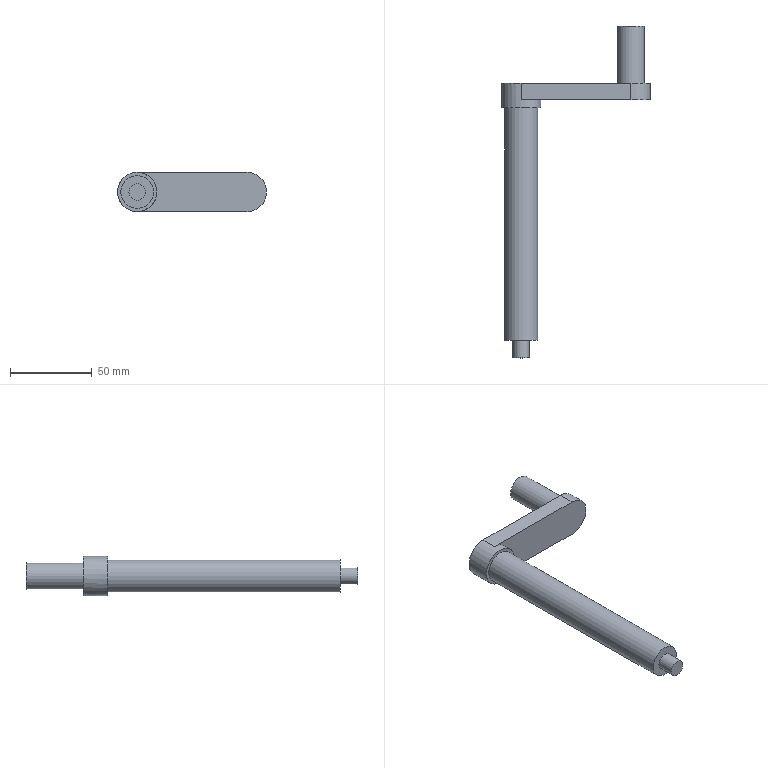Component | NX | ROCKER | 1 solid | 13 faces | box 91 x 202.7 x 24 mm | volume 75353 mm3 | plane 8 | cylinder 5 | commonest cylinder face diameters 24 x2 10 x1 20 x1 16 x1
STEP:
#1=CARTESIAN_POINT('',(0.,0.,0.));
#2=DIRECTION('',(0.,0.,1.));
#3=DIRECTION('',(1.,0.,0.));
#4=AXIS2_PLACEMENT_3D('',#1,#2,#3);
#5=CARTESIAN_POINT('',(-114.826,125.,90.));
#6=VERTEX_POINT('',#5);
#7=CARTESIAN_POINT('',(-126.826,125.,102.));
#8=VERTEX_POINT('',#7);
#9=CARTESIAN_POINT('',(-126.826,125.,90.));
#10=DIRECTION('',(0.,1.,0.));
#11=DIRECTION('',(1.,0.,0.));
#12=AXIS2_PLACEMENT_3D('',#9,#10,#11);
#13=CIRCLE('',#12,12.);
#14=CARTESIAN_POINT('',(-126.826,139.995,90.));
#15=DIRECTION('',(0.,-1.,0.));
#16=DIRECTION('',(-1.,0.,0.));
#17=AXIS2_PLACEMENT_3D('',#14,#15,#16);
#18=CYLINDRICAL_SURFACE('',#17,12.);
#19=CARTESIAN_POINT('',(9.425,14.995));
#20=DIRECTION('',(-1.,0.));
#21=VECTOR('',#20,1.);
#22=LINE('',#19,#21);
#23=(GEOMETRIC_REPRESENTATION_CONTEXT(2)PARAMETRIC_REPRESENTATION_CONTEXT()REPRESENTATION_CONTEXT('',''));
#24=DEFINITIONAL_REPRESENTATION('',(#22),#23);
#25=PCURVE('',#18,#24);
#26=CARTESIAN_POINT('',(-126.826,125.,90.));
#27=DIRECTION('',(0.,1.,0.));
#28=DIRECTION('',(1.,0.,0.));
#29=AXIS2_PLACEMENT_3D('',#26,#27,#28);
#30=PLANE('',#29);
#31=CARTESIAN_POINT('',(0.,0.));
#32=DIRECTION('',(1.,0.));
#33=AXIS2_PLACEMENT_2D('',#31,#32);
#34=CIRCLE('',#33,12.);
#35=(GEOMETRIC_REPRESENTATION_CONTEXT(2)PARAMETRIC_REPRESENTATION_CONTEXT()REPRESENTATION_CONTEXT('',''));
#36=DEFINITIONAL_REPRESENTATION('',(#34),#35);
#37=PCURVE('',#30,#36);
#38=SURFACE_CURVE('',#13,(#25,#37),.PCURVE_S1.);
#39=EDGE_CURVE('',#6,#8,#38,.T.);
#40=ORIENTED_EDGE('',*,*,#39,.T.);
#41=CARTESIAN_POINT('',(-126.826,129.995,102.));
#42=VERTEX_POINT('',#41);
#43=CARTESIAN_POINT('',(-126.826,129.995,102.));
#44=CARTESIAN_POINT('',(-126.826,125.,102.));
#45=B_SPLINE_CURVE_WITH_KNOTS('',1,(#43,#44),.UNSPECIFIED.,.F.,.F.,(2,2),(10.,14.995),.PIECEWISE_BEZIER_KNOTS.);
#46=CARTESIAN_POINT('',(4.712,0.));
#47=DIRECTION('',(0.,1.));
#48=VECTOR('',#47,1.);
#49=LINE('',#46,#48);
#50=(GEOMETRIC_REPRESENTATION_CONTEXT(2)PARAMETRIC_REPRESENTATION_CONTEXT()REPRESENTATION_CONTEXT('',''));
#51=DEFINITIONAL_REPRESENTATION('',(#49),#50);
#52=PCURVE('',#18,#51);
#53=CARTESIAN_POINT('',(10.996,0.));
#54=DIRECTION('',(0.,1.));
#55=VECTOR('',#54,1.);
#56=LINE('',#53,#55);
#57=(GEOMETRIC_REPRESENTATION_CONTEXT(2)PARAMETRIC_REPRESENTATION_CONTEXT()REPRESENTATION_CONTEXT('',''));
#58=DEFINITIONAL_REPRESENTATION('',(#56),#57);
#59=PCURVE('',#18,#58);
#60=SEAM_CURVE('',#45,(#52,#59),.PCURVE_S1.);
#61=EDGE_CURVE('',#42,#8,#60,.T.);
#62=ORIENTED_EDGE('',*,*,#61,.F.);
#63=CARTESIAN_POINT('',(-126.826,139.995,102.));
#64=VERTEX_POINT('',#63);
#65=CARTESIAN_POINT('',(-126.826,139.995,102.));
#66=DIRECTION('',(0.,-1.,0.));
#67=VECTOR('',#66,1.);
#68=LINE('',#65,#67);
#69=CARTESIAN_POINT('',(4.712,0.));
#70=DIRECTION('',(0.,1.));
#71=VECTOR('',#70,1.);
#72=LINE('',#69,#71);
#73=(GEOMETRIC_REPRESENTATION_CONTEXT(2)PARAMETRIC_REPRESENTATION_CONTEXT()REPRESENTATION_CONTEXT('',''));
#74=DEFINITIONAL_REPRESENTATION('',(#72),#73);
#75=PCURVE('',#18,#74);
#76=CARTESIAN_POINT('',(-126.826,139.995,102.));
#77=DIRECTION('',(0.,0.,-1.));
#78=DIRECTION('',(0.,1.,0.));
#79=AXIS2_PLACEMENT_3D('',#76,#77,#78);
#80=PLANE('',#79);
#81=CARTESIAN_POINT('',(0.,0.));
#82=DIRECTION('',(-1.,0.));
#83=VECTOR('',#82,1.);
#84=LINE('',#81,#83);
#85=(GEOMETRIC_REPRESENTATION_CONTEXT(2)PARAMETRIC_REPRESENTATION_CONTEXT()REPRESENTATION_CONTEXT('',''));
#86=DEFINITIONAL_REPRESENTATION('',(#84),#85);
#87=PCURVE('',#80,#86);
#88=SURFACE_CURVE('',#68,(#75,#87),.PCURVE_S1.);
#89=EDGE_CURVE('',#64,#42,#88,.T.);
#90=ORIENTED_EDGE('',*,*,#89,.F.);
#91=CARTESIAN_POINT('',(-126.826,139.995,78.));
#92=VERTEX_POINT('',#91);
#93=CARTESIAN_POINT('',(-126.826,139.995,90.));
#94=DIRECTION('',(0.,1.,0.));
#95=DIRECTION('',(1.,0.,0.));
#96=AXIS2_PLACEMENT_3D('',#93,#94,#95);
#97=CIRCLE('',#96,12.);
#98=CARTESIAN_POINT('',(9.425,0.));
#99=DIRECTION('',(-1.,0.));
#100=VECTOR('',#99,1.);
#101=LINE('',#98,#100);
#102=(GEOMETRIC_REPRESENTATION_CONTEXT(2)PARAMETRIC_REPRESENTATION_CONTEXT()REPRESENTATION_CONTEXT('',''));
#103=DEFINITIONAL_REPRESENTATION('',(#101),#102);
#104=PCURVE('',#18,#103);
#105=CARTESIAN_POINT('',(-126.826,139.995,90.));
#106=DIRECTION('',(0.,1.,0.));
#107=DIRECTION('',(1.,0.,0.));
#108=AXIS2_PLACEMENT_3D('',#105,#106,#107);
#109=PLANE('',#108);
#110=CARTESIAN_POINT('',(0.,0.));
#111=DIRECTION('',(1.,0.));
#112=AXIS2_PLACEMENT_2D('',#110,#111);
#113=CIRCLE('',#112,12.);
#114=(GEOMETRIC_REPRESENTATION_CONTEXT(2)PARAMETRIC_REPRESENTATION_CONTEXT()REPRESENTATION_CONTEXT('',''));
#115=DEFINITIONAL_REPRESENTATION('',(#113),#114);
#116=PCURVE('',#109,#115);
#117=SURFACE_CURVE('',#97,(#104,#116),.PCURVE_S1.);
#118=EDGE_CURVE('',#92,#64,#117,.T.);
#119=ORIENTED_EDGE('',*,*,#118,.F.);
#120=CARTESIAN_POINT('',(-126.826,129.995,78.));
#121=VERTEX_POINT('',#120);
#122=CARTESIAN_POINT('',(-126.826,139.995,78.));
#123=DIRECTION('',(0.,-1.,0.));
#124=VECTOR('',#123,1.);
#125=LINE('',#122,#124);
#126=CARTESIAN_POINT('',(7.854,0.));
#127=DIRECTION('',(0.,1.));
#128=VECTOR('',#127,1.);
#129=LINE('',#126,#128);
#130=(GEOMETRIC_REPRESENTATION_CONTEXT(2)PARAMETRIC_REPRESENTATION_CONTEXT()REPRESENTATION_CONTEXT('',''));
#131=DEFINITIONAL_REPRESENTATION('',(#129),#130);
#132=PCURVE('',#18,#131);
#133=CARTESIAN_POINT('',(-59.827,139.995,78.));
#134=DIRECTION('',(0.,0.,1.));
#135=DIRECTION('',(0.,-1.,0.));
#136=AXIS2_PLACEMENT_3D('',#133,#134,#135);
#137=PLANE('',#136);
#138=CARTESIAN_POINT('',(0.,-67.));
#139=DIRECTION('',(1.,0.));
#140=VECTOR('',#139,1.);
#141=LINE('',#138,#140);
#142=(GEOMETRIC_REPRESENTATION_CONTEXT(2)PARAMETRIC_REPRESENTATION_CONTEXT()REPRESENTATION_CONTEXT('',''));
#143=DEFINITIONAL_REPRESENTATION('',(#141),#142);
#144=PCURVE('',#137,#143);
#145=SURFACE_CURVE('',#125,(#132,#144),.PCURVE_S1.);
#146=EDGE_CURVE('',#92,#121,#145,.T.);
#147=ORIENTED_EDGE('',*,*,#146,.T.);
#148=CARTESIAN_POINT('',(-126.826,129.995,90.));
#149=DIRECTION('',(0.,-1.,0.));
#150=DIRECTION('',(1.,0.,0.));
#151=AXIS2_PLACEMENT_3D('',#148,#149,#150);
#152=CIRCLE('',#151,12.);
#153=CARTESIAN_POINT('',(3.142,10.));
#154=DIRECTION('',(1.,0.));
#155=VECTOR('',#154,1.);
#156=LINE('',#153,#155);
#157=(GEOMETRIC_REPRESENTATION_CONTEXT(2)PARAMETRIC_REPRESENTATION_CONTEXT()REPRESENTATION_CONTEXT('',''));
#158=DEFINITIONAL_REPRESENTATION('',(#156),#157);
#159=PCURVE('',#18,#158);
#160=CARTESIAN_POINT('',(-126.826,129.995,90.));
#161=DIRECTION('',(0.,-1.,0.));
#162=DIRECTION('',(-1.,0.,0.));
#163=AXIS2_PLACEMENT_3D('',#160,#161,#162);
#164=PLANE('',#163);
#165=CARTESIAN_POINT('',(0.,0.));
#166=DIRECTION('',(-1.,0.));
#167=AXIS2_PLACEMENT_2D('',#165,#166);
#168=CIRCLE('',#167,12.);
#169=(GEOMETRIC_REPRESENTATION_CONTEXT(2)PARAMETRIC_REPRESENTATION_CONTEXT()REPRESENTATION_CONTEXT('',''));
#170=DEFINITIONAL_REPRESENTATION('',(#168),#169);
#171=PCURVE('',#164,#170);
#172=SURFACE_CURVE('',#152,(#159,#171),.PCURVE_S1.);
#173=EDGE_CURVE('',#121,#42,#172,.T.);
#174=ORIENTED_EDGE('',*,*,#173,.T.);
#175=ORIENTED_EDGE('',*,*,#61,.T.);
#176=CARTESIAN_POINT('',(-126.826,125.,90.));
#177=DIRECTION('',(0.,1.,0.));
#178=DIRECTION('',(1.,0.,0.));
#179=AXIS2_PLACEMENT_3D('',#176,#177,#178);
#180=CIRCLE('',#179,12.);
#181=CARTESIAN_POINT('',(15.708,14.995));
#182=DIRECTION('',(-1.,0.));
#183=VECTOR('',#182,1.);
#184=LINE('',#181,#183);
#185=(GEOMETRIC_REPRESENTATION_CONTEXT(2)PARAMETRIC_REPRESENTATION_CONTEXT()REPRESENTATION_CONTEXT('',''));
#186=DEFINITIONAL_REPRESENTATION('',(#184),#185);
#187=PCURVE('',#18,#186);
#188=CARTESIAN_POINT('',(0.,0.));
#189=DIRECTION('',(1.,0.));
#190=AXIS2_PLACEMENT_2D('',#188,#189);
#191=CIRCLE('',#190,12.);
#192=(GEOMETRIC_REPRESENTATION_CONTEXT(2)PARAMETRIC_REPRESENTATION_CONTEXT()REPRESENTATION_CONTEXT('',''));
#193=DEFINITIONAL_REPRESENTATION('',(#191),#192);
#194=PCURVE('',#30,#193);
#195=SURFACE_CURVE('',#180,(#187,#194),.PCURVE_S1.);
#196=EDGE_CURVE('',#8,#6,#195,.T.);
#197=ORIENTED_EDGE('',*,*,#196,.T.);
#198=EDGE_LOOP('',(#40,#62,#90,#119,#147,#174,#175,#197));
#199=FACE_BOUND('',#198,.T.);
#200=ADVANCED_FACE('',(#199),#18,.T.);
#201=CARTESIAN_POINT('',(-121.826,-27.705,90.));
#202=VERTEX_POINT('',#201);
#203=CARTESIAN_POINT('',(-126.826,-27.705,90.));
#204=DIRECTION('',(0.,1.,0.));
#205=DIRECTION('',(1.,0.,0.));
#206=AXIS2_PLACEMENT_3D('',#203,#204,#205);
#207=CIRCLE('',#206,5.);
#208=CARTESIAN_POINT('',(-126.826,-27.705,90.));
#209=DIRECTION('',(0.,-1.,0.));
#210=DIRECTION('',(-1.,0.,0.));
#211=AXIS2_PLACEMENT_3D('',#208,#209,#210);
#212=PLANE('',#211);
#213=CARTESIAN_POINT('',(-5.,0.));
#214=CARTESIAN_POINT('',(-5.,8.66));
#215=CARTESIAN_POINT('',(2.5,4.33));
#216=CARTESIAN_POINT('',(10.,0.));
#217=CARTESIAN_POINT('',(2.5,-4.33));
#218=CARTESIAN_POINT('',(-5.,-8.66));
#219=CARTESIAN_POINT('',(-5.,0.));
#220=(BOUNDED_CURVE()B_SPLINE_CURVE(2,(#213,#214,#215,#216,#217,#218,#219),.UNSPECIFIED.,.T.,.F.)B_SPLINE_CURVE_WITH_KNOTS((1,2,2,2,2,1),(-2.094,0.,2.094,4.189,6.283,8.378),.UNSPECIFIED.)CURVE()GEOMETRIC_REPRESENTATION_ITEM()RATIONAL_B_SPLINE_CURVE((1.,0.5,1.,0.5,1.,0.5,1.))REPRESENTATION_ITEM(''));
#221=(GEOMETRIC_REPRESENTATION_CONTEXT(2)PARAMETRIC_REPRESENTATION_CONTEXT()REPRESENTATION_CONTEXT('',''));
#222=DEFINITIONAL_REPRESENTATION('',(#220),#221);
#223=PCURVE('',#212,#222);
#224=CARTESIAN_POINT('',(-126.826,-27.705,90.));
#225=DIRECTION('',(0.,1.,0.));
#226=DIRECTION('',(1.,0.,0.));
#227=AXIS2_PLACEMENT_3D('',#224,#225,#226);
#228=CYLINDRICAL_SURFACE('',#227,5.);
#229=CARTESIAN_POINT('',(0.,0.));
#230=DIRECTION('',(1.,0.));
#231=VECTOR('',#230,1.);
#232=LINE('',#229,#231);
#233=(GEOMETRIC_REPRESENTATION_CONTEXT(2)PARAMETRIC_REPRESENTATION_CONTEXT()REPRESENTATION_CONTEXT('',''));
#234=DEFINITIONAL_REPRESENTATION('',(#232),#233);
#235=PCURVE('',#228,#234);
#236=SURFACE_CURVE('',#207,(#223,#235),.PCURVE_S1.);
#237=EDGE_CURVE('',#202,#202,#236,.T.);
#238=ORIENTED_EDGE('',*,*,#237,.F.);
#239=EDGE_LOOP('',(#238));
#240=FACE_BOUND('',#239,.T.);
#241=ADVANCED_FACE('',(#240),#212,.T.);
#242=CARTESIAN_POINT('',(-121.826,-17.005,90.));
#243=VERTEX_POINT('',#242);
#244=CARTESIAN_POINT('',(-126.826,-17.005,90.));
#245=DIRECTION('',(0.,-1.,0.));
#246=DIRECTION('',(1.,0.,0.));
#247=AXIS2_PLACEMENT_3D('',#244,#245,#246);
#248=CIRCLE('',#247,5.);
#249=CARTESIAN_POINT('',(6.283,10.7));
#250=DIRECTION('',(-1.,0.));
#251=VECTOR('',#250,1.);
#252=LINE('',#249,#251);
#253=(GEOMETRIC_REPRESENTATION_CONTEXT(2)PARAMETRIC_REPRESENTATION_CONTEXT()REPRESENTATION_CONTEXT('',''));
#254=DEFINITIONAL_REPRESENTATION('',(#252),#253);
#255=PCURVE('',#228,#254);
#256=CARTESIAN_POINT('',(-126.826,-17.005,90.));
#257=DIRECTION('',(0.,-1.,0.));
#258=DIRECTION('',(-1.,0.,0.));
#259=AXIS2_PLACEMENT_3D('',#256,#257,#258);
#260=PLANE('',#259);
#261=CARTESIAN_POINT('',(0.,0.));
#262=DIRECTION('',(-1.,0.));
#263=AXIS2_PLACEMENT_2D('',#261,#262);
#264=CIRCLE('',#263,5.);
#265=(GEOMETRIC_REPRESENTATION_CONTEXT(2)PARAMETRIC_REPRESENTATION_CONTEXT()REPRESENTATION_CONTEXT('',''));
#266=DEFINITIONAL_REPRESENTATION('',(#264),#265);
#267=PCURVE('',#260,#266);
#268=SURFACE_CURVE('',#248,(#255,#267),.PCURVE_S1.);
#269=EDGE_CURVE('',#243,#243,#268,.T.);
#270=ORIENTED_EDGE('',*,*,#269,.T.);
#271=CARTESIAN_POINT('',(-121.826,-27.705,90.));
#272=CARTESIAN_POINT('',(-121.826,-17.005,90.));
#273=B_SPLINE_CURVE_WITH_KNOTS('',1,(#271,#272),.UNSPECIFIED.,.F.,.F.,(2,2),(0.,10.7),.PIECEWISE_BEZIER_KNOTS.);
#274=CARTESIAN_POINT('',(0.,0.));
#275=DIRECTION('',(0.,1.));
#276=VECTOR('',#275,1.);
#277=LINE('',#274,#276);
#278=(GEOMETRIC_REPRESENTATION_CONTEXT(2)PARAMETRIC_REPRESENTATION_CONTEXT()REPRESENTATION_CONTEXT('',''));
#279=DEFINITIONAL_REPRESENTATION('',(#277),#278);
#280=PCURVE('',#228,#279);
#281=CARTESIAN_POINT('',(6.283,0.));
#282=DIRECTION('',(0.,1.));
#283=VECTOR('',#282,1.);
#284=LINE('',#281,#283);
#285=(GEOMETRIC_REPRESENTATION_CONTEXT(2)PARAMETRIC_REPRESENTATION_CONTEXT()REPRESENTATION_CONTEXT('',''));
#286=DEFINITIONAL_REPRESENTATION('',(#284),#285);
#287=PCURVE('',#228,#286);
#288=SEAM_CURVE('',#273,(#280,#287),.PCURVE_S1.);
#289=EDGE_CURVE('',#202,#243,#288,.T.);
#290=ORIENTED_EDGE('',*,*,#289,.F.);
#291=ORIENTED_EDGE('',*,*,#237,.T.);
#292=ORIENTED_EDGE('',*,*,#289,.T.);
#293=EDGE_LOOP('',(#270,#290,#291,#292));
#294=FACE_BOUND('',#293,.T.);
#295=ADVANCED_FACE('',(#294),#228,.T.);
#296=ORIENTED_EDGE('',*,*,#269,.F.);
#297=EDGE_LOOP('',(#296));
#298=FACE_BOUND('',#297,.T.);
#299=CARTESIAN_POINT('',(-116.826,-17.005,90.));
#300=VERTEX_POINT('',#299);
#301=CARTESIAN_POINT('',(-126.826,-17.005,90.));
#302=DIRECTION('',(0.,1.,0.));
#303=DIRECTION('',(1.,0.,0.));
#304=AXIS2_PLACEMENT_3D('',#301,#302,#303);
#305=CIRCLE('',#304,10.);
#306=CARTESIAN_POINT('',(-10.,0.));
#307=CARTESIAN_POINT('',(-10.,17.321));
#308=CARTESIAN_POINT('',(5.,8.66));
#309=CARTESIAN_POINT('',(20.,0.));
#310=CARTESIAN_POINT('',(5.,-8.66));
#311=CARTESIAN_POINT('',(-10.,-17.321));
#312=CARTESIAN_POINT('',(-10.,0.));
#313=(BOUNDED_CURVE()B_SPLINE_CURVE(2,(#306,#307,#308,#309,#310,#311,#312),.UNSPECIFIED.,.T.,.F.)B_SPLINE_CURVE_WITH_KNOTS((1,2,2,2,2,1),(-2.094,0.,2.094,4.189,6.283,8.378),.UNSPECIFIED.)CURVE()GEOMETRIC_REPRESENTATION_ITEM()RATIONAL_B_SPLINE_CURVE((1.,0.5,1.,0.5,1.,0.5,1.))REPRESENTATION_ITEM(''));
#314=(GEOMETRIC_REPRESENTATION_CONTEXT(2)PARAMETRIC_REPRESENTATION_CONTEXT()REPRESENTATION_CONTEXT('',''));
#315=DEFINITIONAL_REPRESENTATION('',(#313),#314);
#316=PCURVE('',#260,#315);
#317=CARTESIAN_POINT('',(-126.826,-17.005,90.));
#318=DIRECTION('',(0.,1.,0.));
#319=DIRECTION('',(1.,0.,0.));
#320=AXIS2_PLACEMENT_3D('',#317,#318,#319);
#321=CYLINDRICAL_SURFACE('',#320,10.);
#322=CARTESIAN_POINT('',(0.,0.));
#323=DIRECTION('',(1.,0.));
#324=VECTOR('',#323,1.);
#325=LINE('',#322,#324);
#326=(GEOMETRIC_REPRESENTATION_CONTEXT(2)PARAMETRIC_REPRESENTATION_CONTEXT()REPRESENTATION_CONTEXT('',''));
#327=DEFINITIONAL_REPRESENTATION('',(#325),#326);
#328=PCURVE('',#321,#327);
#329=SURFACE_CURVE('',#305,(#316,#328),.PCURVE_S1.);
#330=EDGE_CURVE('',#300,#300,#329,.T.);
#331=ORIENTED_EDGE('',*,*,#330,.F.);
#332=EDGE_LOOP('',(#331));
#333=FACE_BOUND('',#332,.T.);
#334=ADVANCED_FACE('',(#298,#333),#260,.T.);
#335=CARTESIAN_POINT('',(-116.826,125.,90.));
#336=VERTEX_POINT('',#335);
#337=CARTESIAN_POINT('',(-126.826,125.,90.));
#338=DIRECTION('',(0.,-1.,0.));
#339=DIRECTION('',(1.,0.,0.));
#340=AXIS2_PLACEMENT_3D('',#337,#338,#339);
#341=CIRCLE('',#340,10.);
#342=CARTESIAN_POINT('',(6.283,142.005));
#343=DIRECTION('',(-1.,0.));
#344=VECTOR('',#343,1.);
#345=LINE('',#342,#344);
#346=(GEOMETRIC_REPRESENTATION_CONTEXT(2)PARAMETRIC_REPRESENTATION_CONTEXT()REPRESENTATION_CONTEXT('',''));
#347=DEFINITIONAL_REPRESENTATION('',(#345),#346);
#348=PCURVE('',#321,#347);
#349=CARTESIAN_POINT('',(10.,0.));
#350=CARTESIAN_POINT('',(10.,-17.321));
#351=CARTESIAN_POINT('',(-5.,-8.66));
#352=CARTESIAN_POINT('',(-20.,-0.));
#353=CARTESIAN_POINT('',(-5.,8.66));
#354=CARTESIAN_POINT('',(10.,17.321));
#355=CARTESIAN_POINT('',(10.,0.));
#356=(BOUNDED_CURVE()B_SPLINE_CURVE(2,(#349,#350,#351,#352,#353,#354,#355),.UNSPECIFIED.,.T.,.F.)B_SPLINE_CURVE_WITH_KNOTS((1,2,2,2,2,1),(-2.094,0.,2.094,4.189,6.283,8.378),.UNSPECIFIED.)CURVE()GEOMETRIC_REPRESENTATION_ITEM()RATIONAL_B_SPLINE_CURVE((1.,0.5,1.,0.5,1.,0.5,1.))REPRESENTATION_ITEM(''));
#357=(GEOMETRIC_REPRESENTATION_CONTEXT(2)PARAMETRIC_REPRESENTATION_CONTEXT()REPRESENTATION_CONTEXT('',''));
#358=DEFINITIONAL_REPRESENTATION('',(#356),#357);
#359=PCURVE('',#30,#358);
#360=SURFACE_CURVE('',#341,(#348,#359),.PCURVE_S1.);
#361=EDGE_CURVE('',#336,#336,#360,.T.);
#362=ORIENTED_EDGE('',*,*,#361,.T.);
#363=CARTESIAN_POINT('',(-116.826,-17.005,90.));
#364=CARTESIAN_POINT('',(-116.826,125.,90.));
#365=B_SPLINE_CURVE_WITH_KNOTS('',1,(#363,#364),.UNSPECIFIED.,.F.,.F.,(2,2),(0.,142.005),.PIECEWISE_BEZIER_KNOTS.);
#366=CARTESIAN_POINT('',(0.,0.));
#367=DIRECTION('',(0.,1.));
#368=VECTOR('',#367,1.);
#369=LINE('',#366,#368);
#370=(GEOMETRIC_REPRESENTATION_CONTEXT(2)PARAMETRIC_REPRESENTATION_CONTEXT()REPRESENTATION_CONTEXT('',''));
#371=DEFINITIONAL_REPRESENTATION('',(#369),#370);
#372=PCURVE('',#321,#371);
#373=CARTESIAN_POINT('',(6.283,0.));
#374=DIRECTION('',(0.,1.));
#375=VECTOR('',#374,1.);
#376=LINE('',#373,#375);
#377=(GEOMETRIC_REPRESENTATION_CONTEXT(2)PARAMETRIC_REPRESENTATION_CONTEXT()REPRESENTATION_CONTEXT('',''));
#378=DEFINITIONAL_REPRESENTATION('',(#376),#377);
#379=PCURVE('',#321,#378);
#380=SEAM_CURVE('',#365,(#372,#379),.PCURVE_S1.);
#381=EDGE_CURVE('',#300,#336,#380,.T.);
#382=ORIENTED_EDGE('',*,*,#381,.F.);
#383=ORIENTED_EDGE('',*,*,#330,.T.);
#384=ORIENTED_EDGE('',*,*,#381,.T.);
#385=EDGE_LOOP('',(#362,#382,#383,#384));
#386=FACE_BOUND('',#385,.T.);
#387=ADVANCED_FACE('',(#386),#321,.T.);
#388=CARTESIAN_POINT('',(-51.827,139.995,90.));
#389=VERTEX_POINT('',#388);
#390=CARTESIAN_POINT('',(-59.827,139.995,90.));
#391=DIRECTION('',(0.,1.,0.));
#392=DIRECTION('',(1.,0.,0.));
#393=AXIS2_PLACEMENT_3D('',#390,#391,#392);
#394=CIRCLE('',#393,8.);
#395=CARTESIAN_POINT('',(67.,0.));
#396=DIRECTION('',(1.,0.));
#397=AXIS2_PLACEMENT_2D('',#395,#396);
#398=CIRCLE('',#397,8.);
#399=(GEOMETRIC_REPRESENTATION_CONTEXT(2)PARAMETRIC_REPRESENTATION_CONTEXT()REPRESENTATION_CONTEXT('',''));
#400=DEFINITIONAL_REPRESENTATION('',(#398),#399);
#401=PCURVE('',#109,#400);
#402=CARTESIAN_POINT('',(-59.827,139.995,90.));
#403=DIRECTION('',(0.,1.,0.));
#404=DIRECTION('',(1.,0.,0.));
#405=AXIS2_PLACEMENT_3D('',#402,#403,#404);
#406=CYLINDRICAL_SURFACE('',#405,8.);
#407=CARTESIAN_POINT('',(0.,0.));
#408=DIRECTION('',(1.,0.));
#409=VECTOR('',#408,1.);
#410=LINE('',#407,#409);
#411=(GEOMETRIC_REPRESENTATION_CONTEXT(2)PARAMETRIC_REPRESENTATION_CONTEXT()REPRESENTATION_CONTEXT('',''));
#412=DEFINITIONAL_REPRESENTATION('',(#410),#411);
#413=PCURVE('',#406,#412);
#414=SURFACE_CURVE('',#394,(#401,#413),.PCURVE_S1.);
#415=EDGE_CURVE('',#389,#389,#414,.T.);
#416=ORIENTED_EDGE('',*,*,#415,.F.);
#417=EDGE_LOOP('',(#416));
#418=FACE_BOUND('',#417,.T.);
#419=ORIENTED_EDGE('',*,*,#118,.T.);
#420=CARTESIAN_POINT('',(-59.827,139.995,102.));
#421=VERTEX_POINT('',#420);
#422=CARTESIAN_POINT('',(-126.826,139.995,102.));
#423=DIRECTION('',(1.,0.,0.));
#424=VECTOR('',#423,1.);
#425=LINE('',#422,#424);
#426=CARTESIAN_POINT('',(0.,-12.));
#427=DIRECTION('',(1.,0.));
#428=VECTOR('',#427,1.);
#429=LINE('',#426,#428);
#430=(GEOMETRIC_REPRESENTATION_CONTEXT(2)PARAMETRIC_REPRESENTATION_CONTEXT()REPRESENTATION_CONTEXT('',''));
#431=DEFINITIONAL_REPRESENTATION('',(#429),#430);
#432=PCURVE('',#109,#431);
#433=CARTESIAN_POINT('',(0.,0.));
#434=DIRECTION('',(0.,1.));
#435=VECTOR('',#434,1.);
#436=LINE('',#433,#435);
#437=(GEOMETRIC_REPRESENTATION_CONTEXT(2)PARAMETRIC_REPRESENTATION_CONTEXT()REPRESENTATION_CONTEXT('',''));
#438=DEFINITIONAL_REPRESENTATION('',(#436),#437);
#439=PCURVE('',#80,#438);
#440=SURFACE_CURVE('',#425,(#432,#439),.PCURVE_S1.);
#441=EDGE_CURVE('',#64,#421,#440,.T.);
#442=ORIENTED_EDGE('',*,*,#441,.T.);
#443=CARTESIAN_POINT('',(-59.826,139.995,78.));
#444=VERTEX_POINT('',#443);
#445=CARTESIAN_POINT('',(-59.827,139.995,90.));
#446=DIRECTION('',(0.,1.,0.));
#447=DIRECTION('',(1.,0.,0.));
#448=AXIS2_PLACEMENT_3D('',#445,#446,#447);
#449=CIRCLE('',#448,12.);
#450=CARTESIAN_POINT('',(67.,0.));
#451=DIRECTION('',(1.,0.));
#452=AXIS2_PLACEMENT_2D('',#450,#451);
#453=CIRCLE('',#452,12.);
#454=(GEOMETRIC_REPRESENTATION_CONTEXT(2)PARAMETRIC_REPRESENTATION_CONTEXT()REPRESENTATION_CONTEXT('',''));
#455=DEFINITIONAL_REPRESENTATION('',(#453),#454);
#456=PCURVE('',#109,#455);
#457=CARTESIAN_POINT('',(-59.827,139.995,90.));
#458=DIRECTION('',(0.,-1.,0.));
#459=DIRECTION('',(-1.,0.,0.));
#460=AXIS2_PLACEMENT_3D('',#457,#458,#459);
#461=CYLINDRICAL_SURFACE('',#460,12.);
#462=CARTESIAN_POINT('',(9.425,0.));
#463=DIRECTION('',(-1.,0.));
#464=VECTOR('',#463,1.);
#465=LINE('',#462,#464);
#466=(GEOMETRIC_REPRESENTATION_CONTEXT(2)PARAMETRIC_REPRESENTATION_CONTEXT()REPRESENTATION_CONTEXT('',''));
#467=DEFINITIONAL_REPRESENTATION('',(#465),#466);
#468=PCURVE('',#461,#467);
#469=SURFACE_CURVE('',#449,(#456,#468),.PCURVE_S1.);
#470=EDGE_CURVE('',#421,#444,#469,.T.);
#471=ORIENTED_EDGE('',*,*,#470,.T.);
#472=CARTESIAN_POINT('',(-59.827,139.995,78.));
#473=DIRECTION('',(-1.,0.,0.));
#474=VECTOR('',#473,1.);
#475=LINE('',#472,#474);
#476=CARTESIAN_POINT('',(67.,12.));
#477=DIRECTION('',(-1.,0.));
#478=VECTOR('',#477,1.);
#479=LINE('',#476,#478);
#480=(GEOMETRIC_REPRESENTATION_CONTEXT(2)PARAMETRIC_REPRESENTATION_CONTEXT()REPRESENTATION_CONTEXT('',''));
#481=DEFINITIONAL_REPRESENTATION('',(#479),#480);
#482=PCURVE('',#109,#481);
#483=CARTESIAN_POINT('',(0.,0.));
#484=DIRECTION('',(0.,-1.));
#485=VECTOR('',#484,1.);
#486=LINE('',#483,#485);
#487=(GEOMETRIC_REPRESENTATION_CONTEXT(2)PARAMETRIC_REPRESENTATION_CONTEXT()REPRESENTATION_CONTEXT('',''));
#488=DEFINITIONAL_REPRESENTATION('',(#486),#487);
#489=PCURVE('',#137,#488);
#490=SURFACE_CURVE('',#475,(#482,#489),.PCURVE_S1.);
#491=EDGE_CURVE('',#444,#92,#490,.T.);
#492=ORIENTED_EDGE('',*,*,#491,.T.);
#493=EDGE_LOOP('',(#419,#442,#471,#492));
#494=FACE_BOUND('',#493,.T.);
#495=ADVANCED_FACE('',(#418,#494),#109,.T.);
#496=ORIENTED_EDGE('',*,*,#361,.F.);
#497=EDGE_LOOP('',(#496));
#498=FACE_BOUND('',#497,.T.);
#499=ORIENTED_EDGE('',*,*,#39,.F.);
#500=ORIENTED_EDGE('',*,*,#196,.F.);
#501=EDGE_LOOP('',(#499,#500));
#502=FACE_BOUND('',#501,.T.);
#503=ADVANCED_FACE('',(#498,#502),#30,.F.);
#504=CARTESIAN_POINT('',(-59.827,129.995,102.));
#505=VERTEX_POINT('',#504);
#506=CARTESIAN_POINT('',(-126.826,129.995,102.));
#507=DIRECTION('',(1.,0.,0.));
#508=VECTOR('',#507,1.);
#509=LINE('',#506,#508);
#510=CARTESIAN_POINT('',(-10.,0.));
#511=DIRECTION('',(0.,1.));
#512=VECTOR('',#511,1.);
#513=LINE('',#510,#512);
#514=(GEOMETRIC_REPRESENTATION_CONTEXT(2)PARAMETRIC_REPRESENTATION_CONTEXT()REPRESENTATION_CONTEXT('',''));
#515=DEFINITIONAL_REPRESENTATION('',(#513),#514);
#516=PCURVE('',#80,#515);
#517=CARTESIAN_POINT('',(0.,-12.));
#518=DIRECTION('',(-1.,0.));
#519=VECTOR('',#518,1.);
#520=LINE('',#517,#519);
#521=(GEOMETRIC_REPRESENTATION_CONTEXT(2)PARAMETRIC_REPRESENTATION_CONTEXT()REPRESENTATION_CONTEXT('',''));
#522=DEFINITIONAL_REPRESENTATION('',(#520),#521);
#523=PCURVE('',#164,#522);
#524=SURFACE_CURVE('',#509,(#516,#523),.PCURVE_S1.);
#525=EDGE_CURVE('',#42,#505,#524,.T.);
#526=ORIENTED_EDGE('',*,*,#525,.T.);
#527=CARTESIAN_POINT('',(-59.827,139.995,102.));
#528=DIRECTION('',(0.,-1.,0.));
#529=VECTOR('',#528,1.);
#530=LINE('',#527,#529);
#531=CARTESIAN_POINT('',(0.,67.));
#532=DIRECTION('',(-1.,0.));
#533=VECTOR('',#532,1.);
#534=LINE('',#531,#533);
#535=(GEOMETRIC_REPRESENTATION_CONTEXT(2)PARAMETRIC_REPRESENTATION_CONTEXT()REPRESENTATION_CONTEXT('',''));
#536=DEFINITIONAL_REPRESENTATION('',(#534),#535);
#537=PCURVE('',#80,#536);
#538=CARTESIAN_POINT('',(4.712,0.));
#539=DIRECTION('',(0.,1.));
#540=VECTOR('',#539,1.);
#541=LINE('',#538,#540);
#542=(GEOMETRIC_REPRESENTATION_CONTEXT(2)PARAMETRIC_REPRESENTATION_CONTEXT()REPRESENTATION_CONTEXT('',''));
#543=DEFINITIONAL_REPRESENTATION('',(#541),#542);
#544=PCURVE('',#461,#543);
#545=SURFACE_CURVE('',#530,(#537,#544),.PCURVE_S1.);
#546=EDGE_CURVE('',#421,#505,#545,.T.);
#547=ORIENTED_EDGE('',*,*,#546,.F.);
#548=ORIENTED_EDGE('',*,*,#441,.F.);
#549=ORIENTED_EDGE('',*,*,#89,.T.);
#550=EDGE_LOOP('',(#526,#547,#548,#549));
#551=FACE_BOUND('',#550,.T.);
#552=ADVANCED_FACE('',(#551),#80,.F.);
#553=CARTESIAN_POINT('',(-59.826,129.995,78.));
#554=VERTEX_POINT('',#553);
#555=CARTESIAN_POINT('',(-59.827,129.995,90.));
#556=DIRECTION('',(0.,1.,0.));
#557=DIRECTION('',(1.,0.,0.));
#558=AXIS2_PLACEMENT_3D('',#555,#556,#557);
#559=CIRCLE('',#558,12.);
#560=CARTESIAN_POINT('',(9.425,10.));
#561=DIRECTION('',(-1.,0.));
#562=VECTOR('',#561,1.);
#563=LINE('',#560,#562);
#564=(GEOMETRIC_REPRESENTATION_CONTEXT(2)PARAMETRIC_REPRESENTATION_CONTEXT()REPRESENTATION_CONTEXT('',''));
#565=DEFINITIONAL_REPRESENTATION('',(#563),#564);
#566=PCURVE('',#461,#565);
#567=CARTESIAN_POINT('',(-79.,0.));
#568=CARTESIAN_POINT('',(-79.,20.785));
#569=CARTESIAN_POINT('',(-61.,10.392));
#570=CARTESIAN_POINT('',(-43.,0.));
#571=CARTESIAN_POINT('',(-61.,-10.392));
#572=CARTESIAN_POINT('',(-79.,-20.785));
#573=CARTESIAN_POINT('',(-79.,0.));
#574=(BOUNDED_CURVE()B_SPLINE_CURVE(2,(#567,#568,#569,#570,#571,#572,#573),.UNSPECIFIED.,.T.,.F.)B_SPLINE_CURVE_WITH_KNOTS((1,2,2,2,2,1),(-2.094,0.,2.094,4.189,6.283,8.378),.UNSPECIFIED.)CURVE()GEOMETRIC_REPRESENTATION_ITEM()RATIONAL_B_SPLINE_CURVE((1.,0.5,1.,0.5,1.,0.5,1.))REPRESENTATION_ITEM(''));
#575=(GEOMETRIC_REPRESENTATION_CONTEXT(2)PARAMETRIC_REPRESENTATION_CONTEXT()REPRESENTATION_CONTEXT('',''));
#576=DEFINITIONAL_REPRESENTATION('',(#574),#575);
#577=PCURVE('',#164,#576);
#578=SURFACE_CURVE('',#559,(#566,#577),.PCURVE_S1.);
#579=EDGE_CURVE('',#505,#554,#578,.T.);
#580=ORIENTED_EDGE('',*,*,#579,.T.);
#581=CARTESIAN_POINT('',(-59.826,139.995,78.));
#582=DIRECTION('',(0.,-1.,0.));
#583=VECTOR('',#582,1.);
#584=LINE('',#581,#583);
#585=CARTESIAN_POINT('',(1.571,0.));
#586=DIRECTION('',(0.,1.));
#587=VECTOR('',#586,1.);
#588=LINE('',#585,#587);
#589=(GEOMETRIC_REPRESENTATION_CONTEXT(2)PARAMETRIC_REPRESENTATION_CONTEXT()REPRESENTATION_CONTEXT('',''));
#590=DEFINITIONAL_REPRESENTATION('',(#588),#589);
#591=PCURVE('',#461,#590);
#592=CARTESIAN_POINT('',(0.,0.));
#593=DIRECTION('',(1.,0.));
#594=VECTOR('',#593,1.);
#595=LINE('',#592,#594);
#596=(GEOMETRIC_REPRESENTATION_CONTEXT(2)PARAMETRIC_REPRESENTATION_CONTEXT()REPRESENTATION_CONTEXT('',''));
#597=DEFINITIONAL_REPRESENTATION('',(#595),#596);
#598=PCURVE('',#137,#597);
#599=SURFACE_CURVE('',#584,(#591,#598),.PCURVE_S1.);
#600=EDGE_CURVE('',#444,#554,#599,.T.);
#601=ORIENTED_EDGE('',*,*,#600,.F.);
#602=ORIENTED_EDGE('',*,*,#470,.F.);
#603=ORIENTED_EDGE('',*,*,#546,.T.);
#604=EDGE_LOOP('',(#580,#601,#602,#603));
#605=FACE_BOUND('',#604,.T.);
#606=ADVANCED_FACE('',(#605),#461,.T.);
#607=CARTESIAN_POINT('',(-59.827,129.995,78.));
#608=DIRECTION('',(-1.,0.,0.));
#609=VECTOR('',#608,1.);
#610=LINE('',#607,#609);
#611=CARTESIAN_POINT('',(10.,0.));
#612=DIRECTION('',(0.,-1.));
#613=VECTOR('',#612,1.);
#614=LINE('',#611,#613);
#615=(GEOMETRIC_REPRESENTATION_CONTEXT(2)PARAMETRIC_REPRESENTATION_CONTEXT()REPRESENTATION_CONTEXT('',''));
#616=DEFINITIONAL_REPRESENTATION('',(#614),#615);
#617=PCURVE('',#137,#616);
#618=CARTESIAN_POINT('',(-67.,12.));
#619=DIRECTION('',(1.,0.));
#620=VECTOR('',#619,1.);
#621=LINE('',#618,#620);
#622=(GEOMETRIC_REPRESENTATION_CONTEXT(2)PARAMETRIC_REPRESENTATION_CONTEXT()REPRESENTATION_CONTEXT('',''));
#623=DEFINITIONAL_REPRESENTATION('',(#621),#622);
#624=PCURVE('',#164,#623);
#625=SURFACE_CURVE('',#610,(#617,#624),.PCURVE_S1.);
#626=EDGE_CURVE('',#554,#121,#625,.T.);
#627=ORIENTED_EDGE('',*,*,#626,.T.);
#628=ORIENTED_EDGE('',*,*,#146,.F.);
#629=ORIENTED_EDGE('',*,*,#491,.F.);
#630=ORIENTED_EDGE('',*,*,#600,.T.);
#631=EDGE_LOOP('',(#627,#628,#629,#630));
#632=FACE_BOUND('',#631,.T.);
#633=ADVANCED_FACE('',(#632),#137,.F.);
#634=ORIENTED_EDGE('',*,*,#173,.F.);
#635=ORIENTED_EDGE('',*,*,#626,.F.);
#636=ORIENTED_EDGE('',*,*,#579,.F.);
#637=ORIENTED_EDGE('',*,*,#525,.F.);
#638=EDGE_LOOP('',(#634,#635,#636,#637));
#639=FACE_BOUND('',#638,.T.);
#640=ADVANCED_FACE('',(#639),#164,.T.);
#641=CARTESIAN_POINT('',(-51.827,174.995,90.));
#642=VERTEX_POINT('',#641);
#643=CARTESIAN_POINT('',(-59.827,174.995,90.));
#644=DIRECTION('',(0.,-1.,0.));
#645=DIRECTION('',(1.,0.,0.));
#646=AXIS2_PLACEMENT_3D('',#643,#644,#645);
#647=CIRCLE('',#646,8.);
#648=CARTESIAN_POINT('',(-59.827,174.995,90.));
#649=DIRECTION('',(0.,1.,0.));
#650=DIRECTION('',(1.,0.,0.));
#651=AXIS2_PLACEMENT_3D('',#648,#649,#650);
#652=PLANE('',#651);
#653=CARTESIAN_POINT('',(8.,0.));
#654=CARTESIAN_POINT('',(8.,-13.856));
#655=CARTESIAN_POINT('',(-4.,-6.928));
#656=CARTESIAN_POINT('',(-16.,-0.));
#657=CARTESIAN_POINT('',(-4.,6.928));
#658=CARTESIAN_POINT('',(8.,13.856));
#659=CARTESIAN_POINT('',(8.,0.));
#660=(BOUNDED_CURVE()B_SPLINE_CURVE(2,(#653,#654,#655,#656,#657,#658,#659),.UNSPECIFIED.,.T.,.F.)B_SPLINE_CURVE_WITH_KNOTS((1,2,2,2,2,1),(-2.094,0.,2.094,4.189,6.283,8.378),.UNSPECIFIED.)CURVE()GEOMETRIC_REPRESENTATION_ITEM()RATIONAL_B_SPLINE_CURVE((1.,0.5,1.,0.5,1.,0.5,1.))REPRESENTATION_ITEM(''));
#661=(GEOMETRIC_REPRESENTATION_CONTEXT(2)PARAMETRIC_REPRESENTATION_CONTEXT()REPRESENTATION_CONTEXT('',''));
#662=DEFINITIONAL_REPRESENTATION('',(#660),#661);
#663=PCURVE('',#652,#662);
#664=CARTESIAN_POINT('',(6.283,35.));
#665=DIRECTION('',(-1.,0.));
#666=VECTOR('',#665,1.);
#667=LINE('',#664,#666);
#668=(GEOMETRIC_REPRESENTATION_CONTEXT(2)PARAMETRIC_REPRESENTATION_CONTEXT()REPRESENTATION_CONTEXT('',''));
#669=DEFINITIONAL_REPRESENTATION('',(#667),#668);
#670=PCURVE('',#406,#669);
#671=SURFACE_CURVE('',#647,(#663,#670),.PCURVE_S1.);
#672=EDGE_CURVE('',#642,#642,#671,.T.);
#673=ORIENTED_EDGE('',*,*,#672,.F.);
#674=EDGE_LOOP('',(#673));
#675=FACE_BOUND('',#674,.T.);
#676=ADVANCED_FACE('',(#675),#652,.T.);
#677=ORIENTED_EDGE('',*,*,#672,.T.);
#678=CARTESIAN_POINT('',(-51.827,139.995,90.));
#679=CARTESIAN_POINT('',(-51.827,174.995,90.));
#680=B_SPLINE_CURVE_WITH_KNOTS('',1,(#678,#679),.UNSPECIFIED.,.F.,.F.,(2,2),(0.,35.),.PIECEWISE_BEZIER_KNOTS.);
#681=CARTESIAN_POINT('',(0.,0.));
#682=DIRECTION('',(0.,1.));
#683=VECTOR('',#682,1.);
#684=LINE('',#681,#683);
#685=(GEOMETRIC_REPRESENTATION_CONTEXT(2)PARAMETRIC_REPRESENTATION_CONTEXT()REPRESENTATION_CONTEXT('',''));
#686=DEFINITIONAL_REPRESENTATION('',(#684),#685);
#687=PCURVE('',#406,#686);
#688=CARTESIAN_POINT('',(6.283,0.));
#689=DIRECTION('',(0.,1.));
#690=VECTOR('',#689,1.);
#691=LINE('',#688,#690);
#692=(GEOMETRIC_REPRESENTATION_CONTEXT(2)PARAMETRIC_REPRESENTATION_CONTEXT()REPRESENTATION_CONTEXT('',''));
#693=DEFINITIONAL_REPRESENTATION('',(#691),#692);
#694=PCURVE('',#406,#693);
#695=SEAM_CURVE('',#680,(#687,#694),.PCURVE_S1.);
#696=EDGE_CURVE('',#389,#642,#695,.T.);
#697=ORIENTED_EDGE('',*,*,#696,.F.);
#698=ORIENTED_EDGE('',*,*,#415,.T.);
#699=ORIENTED_EDGE('',*,*,#696,.T.);
#700=EDGE_LOOP('',(#677,#697,#698,#699));
#701=FACE_BOUND('',#700,.T.);
#702=ADVANCED_FACE('',(#701),#406,.T.);
#703=CLOSED_SHELL('',(#200,#241,#295,#334,#387,#495,#503,#552,#606,#633,#640,#676,#702));
#704=MANIFOLD_SOLID_BREP('',#703);
#705=(LENGTH_UNIT()NAMED_UNIT(*)SI_UNIT(.MILLI.,.METRE.));
#706=UNCERTAINTY_MEASURE_WITH_UNIT(LENGTH_MEASURE(0.000005),#705,'','');
#707=(NAMED_UNIT(*)PLANE_ANGLE_UNIT()SI_UNIT($,.RADIAN.));
#708=(NAMED_UNIT(*)SI_UNIT($,.STERADIAN.)SOLID_ANGLE_UNIT());
#709=(GEOMETRIC_REPRESENTATION_CONTEXT(3)GLOBAL_UNCERTAINTY_ASSIGNED_CONTEXT((#706))GLOBAL_UNIT_ASSIGNED_CONTEXT((#705,#707,#708))REPRESENTATION_CONTEXT('',''));
#710=ADVANCED_BREP_SHAPE_REPRESENTATION('',(#4,#704),#709);